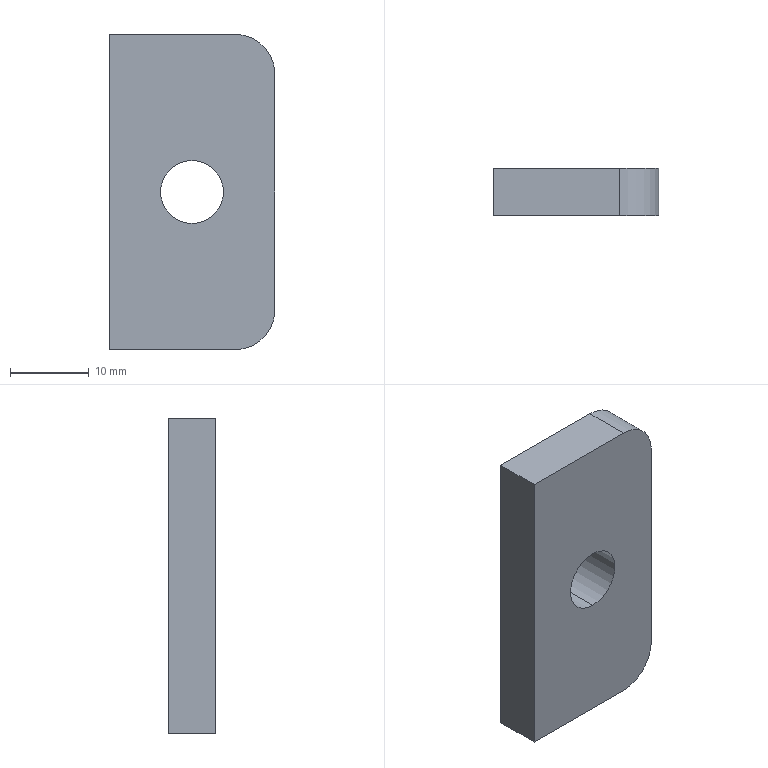Component | SolidWorks | BeltLineSidePlate-1_YL1.sldasm-Part-85-1 | 1 solid | 10 faces | box 21 x 6 x 40 mm | volume 4674 mm3 | plane 6 | cylinder 4 | commonest cylinder face diameters 8 x2 10 x2
STEP:
#1=COLOUR_RGB('',0.7922,0.8196,0.9333);
#2=FILL_AREA_STYLE_COLOUR('',#1);
#3=FILL_AREA_STYLE('',(#2));
#4=SURFACE_STYLE_FILL_AREA(#3);
#5=SURFACE_SIDE_STYLE('',(#4));
#6=SURFACE_STYLE_USAGE(.BOTH.,#5);
#7=PRESENTATION_STYLE_ASSIGNMENT((#6));
#8=CARTESIAN_POINT('',(240.374,117.94,2.023));
#9=VERTEX_POINT('',#8);
#10=CARTESIAN_POINT('',(240.374,117.94,1.708));
#11=VERTEX_POINT('',#10);
#12=CARTESIAN_POINT('',(240.374,117.94,1.865));
#13=DIRECTION('',(0.,1.,0.));
#14=DIRECTION('',(0.,0.,1.));
#15=AXIS2_PLACEMENT_3D('',#12,#13,#14);
#16=CIRCLE('',#15,0.1575);
#17=EDGE_CURVE('',#9,#11,#16,.T.);
#18=ORIENTED_EDGE('',*,*,#17,.T.);
#19=CARTESIAN_POINT('',(240.374,117.704,1.708));
#20=VERTEX_POINT('',#19);
#21=CARTESIAN_POINT('',(240.374,119.2,1.708));
#22=DIRECTION('',(-0.,-1.,-0.));
#23=VECTOR('',#22,39.37);
#24=LINE('',#21,#23);
#25=EDGE_CURVE('',#11,#20,#24,.T.);
#26=ORIENTED_EDGE('',*,*,#25,.T.);
#27=CARTESIAN_POINT('',(240.374,117.704,2.023));
#28=VERTEX_POINT('',#27);
#29=CARTESIAN_POINT('',(240.374,117.704,1.865));
#30=DIRECTION('',(-0.,-1.,-0.));
#31=DIRECTION('',(0.,0.,-1.));
#32=AXIS2_PLACEMENT_3D('',#29,#30,#31);
#33=CIRCLE('',#32,0.1575);
#34=EDGE_CURVE('',#20,#28,#33,.T.);
#35=ORIENTED_EDGE('',*,*,#34,.T.);
#36=CARTESIAN_POINT('',(240.374,119.2,2.023));
#37=DIRECTION('',(-0.,-1.,-0.));
#38=VECTOR('',#37,39.37);
#39=LINE('',#36,#38);
#40=EDGE_CURVE('',#9,#28,#39,.T.);
#41=ORIENTED_EDGE('',*,*,#40,.F.);
#42=EDGE_LOOP('',(#18,#26,#35,#41));
#43=FACE_OUTER_BOUND('',#42,.T.);
#44=CARTESIAN_POINT('',(240.374,119.2,1.865));
#45=DIRECTION('',(-0.,-1.,-0.));
#46=DIRECTION('',(0.,0.,1.));
#47=AXIS2_PLACEMENT_3D('',#44,#45,#46);
#48=CYLINDRICAL_SURFACE('',#47,0.1575);
#49=ADVANCED_FACE('',(#43),#48,.F.);
#50=CARTESIAN_POINT('',(240.591,117.94,2.653));
#51=VERTEX_POINT('',#50);
#52=CARTESIAN_POINT('',(239.961,117.94,2.653));
#53=VERTEX_POINT('',#52);
#54=CARTESIAN_POINT('',(240.788,117.94,2.653));
#55=DIRECTION('',(-1.,0.,0.));
#56=VECTOR('',#55,39.37);
#57=LINE('',#54,#56);
#58=EDGE_CURVE('',#51,#53,#57,.T.);
#59=ORIENTED_EDGE('',*,*,#58,.T.);
#60=CARTESIAN_POINT('',(239.961,117.704,2.653));
#61=VERTEX_POINT('',#60);
#62=CARTESIAN_POINT('',(239.961,117.704,2.653));
#63=DIRECTION('',(0.,1.,0.));
#64=VECTOR('',#63,39.37);
#65=LINE('',#62,#64);
#66=EDGE_CURVE('',#61,#53,#65,.T.);
#67=ORIENTED_EDGE('',*,*,#66,.F.);
#68=CARTESIAN_POINT('',(240.591,117.704,2.653));
#69=VERTEX_POINT('',#68);
#70=CARTESIAN_POINT('',(240.788,117.704,2.653));
#71=DIRECTION('',(-1.,0.,0.));
#72=VECTOR('',#71,39.37);
#73=LINE('',#70,#72);
#74=EDGE_CURVE('',#69,#61,#73,.T.);
#75=ORIENTED_EDGE('',*,*,#74,.F.);
#76=CARTESIAN_POINT('',(240.591,117.704,2.653));
#77=DIRECTION('',(-0.,-1.,-0.));
#78=VECTOR('',#77,39.37);
#79=LINE('',#76,#78);
#80=EDGE_CURVE('',#51,#69,#79,.T.);
#81=ORIENTED_EDGE('',*,*,#80,.F.);
#82=EDGE_LOOP('',(#59,#67,#75,#81));
#83=FACE_OUTER_BOUND('',#82,.T.);
#84=CARTESIAN_POINT('',(240.788,117.704,2.653));
#85=DIRECTION('',(0.,0.,-1.));
#86=DIRECTION('',(-0.,-1.,-0.));
#87=AXIS2_PLACEMENT_3D('',#84,#85,#86);
#88=PLANE('',#87);
#89=ADVANCED_FACE('',(#83),#88,.F.);
#90=ORIENTED_EDGE('',*,*,#17,.F.);
#91=CARTESIAN_POINT('',(240.374,117.94,1.865));
#92=DIRECTION('',(0.,1.,0.));
#93=DIRECTION('',(0.,0.,1.));
#94=AXIS2_PLACEMENT_3D('',#91,#92,#93);
#95=CIRCLE('',#94,0.1575);
#96=EDGE_CURVE('',#11,#9,#95,.T.);
#97=ORIENTED_EDGE('',*,*,#96,.F.);
#98=EDGE_LOOP('',(#90,#97));
#99=FACE_BOUND('',#98,.T.);
#100=CARTESIAN_POINT('',(240.591,117.94,1.078));
#101=VERTEX_POINT('',#100);
#102=CARTESIAN_POINT('',(239.961,117.94,1.078));
#103=VERTEX_POINT('',#102);
#104=CARTESIAN_POINT('',(240.788,117.94,1.078));
#105=DIRECTION('',(-1.,0.,0.));
#106=VECTOR('',#105,39.37);
#107=LINE('',#104,#106);
#108=EDGE_CURVE('',#101,#103,#107,.T.);
#109=ORIENTED_EDGE('',*,*,#108,.T.);
#110=CARTESIAN_POINT('',(239.961,117.94,2.653));
#111=DIRECTION('',(0.,0.,-1.));
#112=VECTOR('',#111,39.37);
#113=LINE('',#110,#112);
#114=EDGE_CURVE('',#53,#103,#113,.T.);
#115=ORIENTED_EDGE('',*,*,#114,.F.);
#116=ORIENTED_EDGE('',*,*,#58,.F.);
#117=CARTESIAN_POINT('',(240.788,117.94,2.456));
#118=VERTEX_POINT('',#117);
#119=CARTESIAN_POINT('',(240.591,117.94,2.456));
#120=DIRECTION('',(-0.,-1.,-0.));
#121=DIRECTION('',(0.,0.,1.));
#122=AXIS2_PLACEMENT_3D('',#119,#120,#121);
#123=CIRCLE('',#122,0.1969);
#124=EDGE_CURVE('',#118,#51,#123,.T.);
#125=ORIENTED_EDGE('',*,*,#124,.F.);
#126=CARTESIAN_POINT('',(240.788,117.94,1.275));
#127=VERTEX_POINT('',#126);
#128=CARTESIAN_POINT('',(240.788,117.94,2.653));
#129=DIRECTION('',(0.,0.,-1.));
#130=VECTOR('',#129,39.37);
#131=LINE('',#128,#130);
#132=EDGE_CURVE('',#118,#127,#131,.T.);
#133=ORIENTED_EDGE('',*,*,#132,.T.);
#134=CARTESIAN_POINT('',(240.591,117.94,1.275));
#135=DIRECTION('',(-0.,-1.,-0.));
#136=DIRECTION('',(0.,0.,1.));
#137=AXIS2_PLACEMENT_3D('',#134,#135,#136);
#138=CIRCLE('',#137,0.1969);
#139=EDGE_CURVE('',#101,#127,#138,.T.);
#140=ORIENTED_EDGE('',*,*,#139,.F.);
#141=EDGE_LOOP('',(#109,#115,#116,#125,#133,#140));
#142=FACE_OUTER_BOUND('',#141,.T.);
#143=CARTESIAN_POINT('',(240.788,117.94,2.653));
#144=DIRECTION('',(-0.,-1.,-0.));
#145=DIRECTION('',(-0.,-0.,1.));
#146=AXIS2_PLACEMENT_3D('',#143,#144,#145);
#147=PLANE('',#146);
#148=ADVANCED_FACE('',(#99,#142),#147,.F.);
#149=CARTESIAN_POINT('',(240.591,117.704,1.078));
#150=VERTEX_POINT('',#149);
#151=CARTESIAN_POINT('',(239.961,117.704,1.078));
#152=VERTEX_POINT('',#151);
#153=CARTESIAN_POINT('',(240.788,117.704,1.078));
#154=DIRECTION('',(-1.,0.,0.));
#155=VECTOR('',#154,39.37);
#156=LINE('',#153,#155);
#157=EDGE_CURVE('',#150,#152,#156,.T.);
#158=ORIENTED_EDGE('',*,*,#157,.T.);
#159=CARTESIAN_POINT('',(239.961,117.94,1.078));
#160=DIRECTION('',(-0.,-1.,-0.));
#161=VECTOR('',#160,39.37);
#162=LINE('',#159,#161);
#163=EDGE_CURVE('',#103,#152,#162,.T.);
#164=ORIENTED_EDGE('',*,*,#163,.F.);
#165=ORIENTED_EDGE('',*,*,#108,.F.);
#166=CARTESIAN_POINT('',(240.591,117.94,1.078));
#167=DIRECTION('',(0.,1.,0.));
#168=VECTOR('',#167,39.37);
#169=LINE('',#166,#168);
#170=EDGE_CURVE('',#150,#101,#169,.T.);
#171=ORIENTED_EDGE('',*,*,#170,.F.);
#172=EDGE_LOOP('',(#158,#164,#165,#171));
#173=FACE_OUTER_BOUND('',#172,.T.);
#174=CARTESIAN_POINT('',(240.788,117.94,1.078));
#175=DIRECTION('',(-0.,-0.,1.));
#176=DIRECTION('',(0.,1.,0.));
#177=AXIS2_PLACEMENT_3D('',#174,#175,#176);
#178=PLANE('',#177);
#179=ADVANCED_FACE('',(#173),#178,.F.);
#180=CARTESIAN_POINT('',(240.374,117.704,1.865));
#181=DIRECTION('',(-0.,-1.,-0.));
#182=DIRECTION('',(0.,0.,-1.));
#183=AXIS2_PLACEMENT_3D('',#180,#181,#182);
#184=CIRCLE('',#183,0.1575);
#185=EDGE_CURVE('',#28,#20,#184,.T.);
#186=ORIENTED_EDGE('',*,*,#185,.F.);
#187=ORIENTED_EDGE('',*,*,#34,.F.);
#188=EDGE_LOOP('',(#186,#187));
#189=FACE_BOUND('',#188,.T.);
#190=CARTESIAN_POINT('',(240.788,117.704,1.275));
#191=VERTEX_POINT('',#190);
#192=CARTESIAN_POINT('',(240.788,117.704,2.456));
#193=VERTEX_POINT('',#192);
#194=CARTESIAN_POINT('',(240.788,117.704,1.078));
#195=DIRECTION('',(-0.,-0.,1.));
#196=VECTOR('',#195,39.37);
#197=LINE('',#194,#196);
#198=EDGE_CURVE('',#191,#193,#197,.T.);
#199=ORIENTED_EDGE('',*,*,#198,.T.);
#200=CARTESIAN_POINT('',(240.591,117.704,2.456));
#201=DIRECTION('',(0.,1.,0.));
#202=DIRECTION('',(0.,0.,-1.));
#203=AXIS2_PLACEMENT_3D('',#200,#201,#202);
#204=CIRCLE('',#203,0.1969);
#205=EDGE_CURVE('',#69,#193,#204,.T.);
#206=ORIENTED_EDGE('',*,*,#205,.F.);
#207=ORIENTED_EDGE('',*,*,#74,.T.);
#208=CARTESIAN_POINT('',(239.961,117.704,1.078));
#209=DIRECTION('',(-0.,-0.,1.));
#210=VECTOR('',#209,39.37);
#211=LINE('',#208,#210);
#212=EDGE_CURVE('',#152,#61,#211,.T.);
#213=ORIENTED_EDGE('',*,*,#212,.F.);
#214=ORIENTED_EDGE('',*,*,#157,.F.);
#215=CARTESIAN_POINT('',(240.591,117.704,1.275));
#216=DIRECTION('',(0.,1.,0.));
#217=DIRECTION('',(0.,0.,-1.));
#218=AXIS2_PLACEMENT_3D('',#215,#216,#217);
#219=CIRCLE('',#218,0.1969);
#220=EDGE_CURVE('',#191,#150,#219,.T.);
#221=ORIENTED_EDGE('',*,*,#220,.F.);
#222=EDGE_LOOP('',(#199,#206,#207,#213,#214,#221));
#223=FACE_OUTER_BOUND('',#222,.T.);
#224=CARTESIAN_POINT('',(240.788,117.704,1.078));
#225=DIRECTION('',(0.,1.,0.));
#226=DIRECTION('',(0.,0.,-1.));
#227=AXIS2_PLACEMENT_3D('',#224,#225,#226);
#228=PLANE('',#227);
#229=ADVANCED_FACE('',(#189,#223),#228,.F.);
#230=ORIENTED_EDGE('',*,*,#132,.F.);
#231=CARTESIAN_POINT('',(240.788,117.94,2.456));
#232=DIRECTION('',(0.,1.,0.));
#233=VECTOR('',#232,39.37);
#234=LINE('',#231,#233);
#235=EDGE_CURVE('',#193,#118,#234,.T.);
#236=ORIENTED_EDGE('',*,*,#235,.F.);
#237=ORIENTED_EDGE('',*,*,#198,.F.);
#238=CARTESIAN_POINT('',(240.788,117.704,1.275));
#239=DIRECTION('',(-0.,-1.,-0.));
#240=VECTOR('',#239,39.37);
#241=LINE('',#238,#240);
#242=EDGE_CURVE('',#127,#191,#241,.T.);
#243=ORIENTED_EDGE('',*,*,#242,.F.);
#244=EDGE_LOOP('',(#230,#236,#237,#243));
#245=FACE_OUTER_BOUND('',#244,.T.);
#246=CARTESIAN_POINT('',(240.788,117.94,2.653));
#247=DIRECTION('',(1.,-0.,-0.));
#248=DIRECTION('',(0.,0.,-1.));
#249=AXIS2_PLACEMENT_3D('',#246,#247,#248);
#250=PLANE('',#249);
#251=ADVANCED_FACE('',(#245),#250,.T.);
#252=ORIENTED_EDGE('',*,*,#66,.T.);
#253=ORIENTED_EDGE('',*,*,#114,.T.);
#254=ORIENTED_EDGE('',*,*,#163,.T.);
#255=ORIENTED_EDGE('',*,*,#212,.T.);
#256=EDGE_LOOP('',(#252,#253,#254,#255));
#257=FACE_OUTER_BOUND('',#256,.T.);
#258=CARTESIAN_POINT('',(239.961,117.94,2.653));
#259=DIRECTION('',(1.,-0.,-0.));
#260=DIRECTION('',(0.,0.,-1.));
#261=AXIS2_PLACEMENT_3D('',#258,#259,#260);
#262=PLANE('',#261);
#263=ADVANCED_FACE('',(#257),#262,.F.);
#264=ORIENTED_EDGE('',*,*,#205,.T.);
#265=ORIENTED_EDGE('',*,*,#235,.T.);
#266=ORIENTED_EDGE('',*,*,#124,.T.);
#267=ORIENTED_EDGE('',*,*,#80,.T.);
#268=EDGE_LOOP('',(#264,#265,#266,#267));
#269=FACE_OUTER_BOUND('',#268,.T.);
#270=CARTESIAN_POINT('',(240.591,117.94,2.456));
#271=DIRECTION('',(-0.,-1.,-0.));
#272=DIRECTION('',(0.,0.,1.));
#273=AXIS2_PLACEMENT_3D('',#270,#271,#272);
#274=CYLINDRICAL_SURFACE('',#273,0.1969);
#275=ADVANCED_FACE('',(#269),#274,.T.);
#276=ORIENTED_EDGE('',*,*,#139,.T.);
#277=ORIENTED_EDGE('',*,*,#242,.T.);
#278=ORIENTED_EDGE('',*,*,#220,.T.);
#279=ORIENTED_EDGE('',*,*,#170,.T.);
#280=EDGE_LOOP('',(#276,#277,#278,#279));
#281=FACE_OUTER_BOUND('',#280,.T.);
#282=CARTESIAN_POINT('',(240.591,117.94,1.275));
#283=DIRECTION('',(0.,1.,0.));
#284=DIRECTION('',(0.,0.,-1.));
#285=AXIS2_PLACEMENT_3D('',#282,#283,#284);
#286=CYLINDRICAL_SURFACE('',#285,0.1969);
#287=ADVANCED_FACE('',(#281),#286,.T.);
#288=ORIENTED_EDGE('',*,*,#25,.F.);
#289=ORIENTED_EDGE('',*,*,#96,.T.);
#290=ORIENTED_EDGE('',*,*,#40,.T.);
#291=ORIENTED_EDGE('',*,*,#185,.T.);
#292=EDGE_LOOP('',(#288,#289,#290,#291));
#293=FACE_OUTER_BOUND('',#292,.T.);
#294=CARTESIAN_POINT('',(240.374,119.2,1.865));
#295=DIRECTION('',(-0.,-1.,-0.));
#296=DIRECTION('',(0.,0.,1.));
#297=AXIS2_PLACEMENT_3D('',#294,#295,#296);
#298=CYLINDRICAL_SURFACE('',#297,0.1575);
#299=ADVANCED_FACE('',(#293),#298,.F.);
#300=CLOSED_SHELL('',(#49,#89,#148,#179,#229,#251,#263,#275,#287,#299));
#301=MANIFOLD_SOLID_BREP('',#300);
#302=STYLED_ITEM('',(#7),#301);
#303=PRESENTATION_LAYER_ASSIGNMENT('','',(#302));
#304=CARTESIAN_POINT('',(0.,0.,0.));
#305=DIRECTION('',(0.,0.,1.));
#306=DIRECTION('',(1.,0.,0.));
#307=AXIS2_PLACEMENT_3D('',#304,#305,#306);
#308=(LENGTH_UNIT()NAMED_UNIT(*)SI_UNIT($,.METRE.));
#309=LENGTH_MEASURE_WITH_UNIT(LENGTH_MEASURE(0.0254),#308);
#310=DIMENSIONAL_EXPONENTS(1.,0.,0.,0.,0.,0.,0.);
#311=(CONVERSION_BASED_UNIT('',#309)LENGTH_UNIT()NAMED_UNIT(#310));
#312=UNCERTAINTY_MEASURE_WITH_UNIT(LENGTH_MEASURE(0.00001),#311,'','');
#313=(NAMED_UNIT(*)PLANE_ANGLE_UNIT()SI_UNIT($,.RADIAN.));
#314=(NAMED_UNIT(*)SI_UNIT($,.STERADIAN.)SOLID_ANGLE_UNIT());
#315=(GEOMETRIC_REPRESENTATION_CONTEXT(3)GLOBAL_UNCERTAINTY_ASSIGNED_CONTEXT((#312))GLOBAL_UNIT_ASSIGNED_CONTEXT((#311,#313,#314))REPRESENTATION_CONTEXT('',''));
#316=ADVANCED_BREP_SHAPE_REPRESENTATION('',(#301,#307),#315);
#317=(LENGTH_UNIT()NAMED_UNIT(*)SI_UNIT($,.METRE.));
#318=LENGTH_MEASURE_WITH_UNIT(LENGTH_MEASURE(0.0254),#317);
#319=DIMENSIONAL_EXPONENTS(1.,0.,0.,0.,0.,0.,0.);
#320=(CONVERSION_BASED_UNIT('',#318)LENGTH_UNIT()NAMED_UNIT(#319));
#321=UNCERTAINTY_MEASURE_WITH_UNIT(LENGTH_MEASURE(0.00001),#320,'','');
#322=(NAMED_UNIT(*)PLANE_ANGLE_UNIT()SI_UNIT($,.RADIAN.));
#323=(NAMED_UNIT(*)SI_UNIT($,.STERADIAN.)SOLID_ANGLE_UNIT());
#324=(GEOMETRIC_REPRESENTATION_CONTEXT(3)GLOBAL_UNCERTAINTY_ASSIGNED_CONTEXT((#321))GLOBAL_UNIT_ASSIGNED_CONTEXT((#320,#322,#323))REPRESENTATION_CONTEXT('',''));
#325=MECHANICAL_DESIGN_GEOMETRIC_PRESENTATION_REPRESENTATION('',(#302),#324);